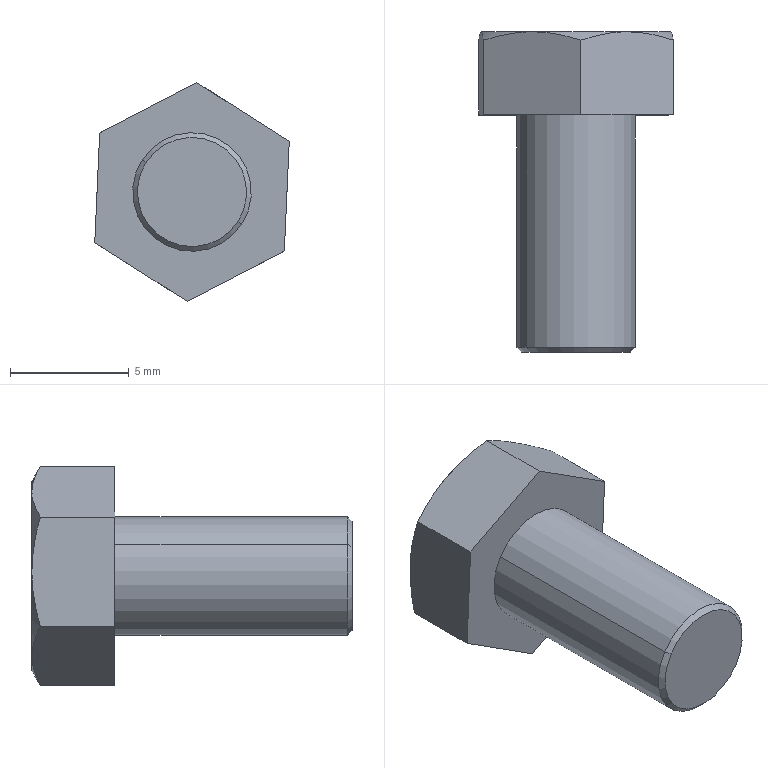Component | SolidWorks | TRCBASHexagonThroughHoleBolt[TRCBAS5-10]-1 | 1 solid | 20 faces | box 8.2 x 13.5 x 9.23 mm | volume 389 mm3 | cone 9 | plane 9 | cylinder 2 | commonest cylinder face diameters 5 x2
STEP:
#1=CARTESIAN_POINT('',(1.307,-10.008,-29.746));
#2=VERTEX_POINT('',#1);
#3=CARTESIAN_POINT('',(1.154,-10.008,-29.648));
#4=VERTEX_POINT('',#3);
#5=CARTESIAN_POINT('',(1.23,-10.008,-29.697));
#6=DIRECTION('',(0.,-1.,0.));
#7=DIRECTION('',(0.8429,0.,-0.5381));
#8=AXIS2_PLACEMENT_3D('',#5,#6,#7);
#9=CIRCLE('',#8,0.09055);
#10=EDGE_CURVE('',#2,#4,#9,.T.);
#11=ORIENTED_EDGE('',*,*,#10,.F.);
#12=CARTESIAN_POINT('',(1.313,-10.,-29.75));
#13=VERTEX_POINT('',#12);
#14=CARTESIAN_POINT('',(1.313,-10.,-29.75));
#15=DIRECTION('',(0.596,0.7071,-0.3805));
#16=VECTOR('',#15,39.37);
#17=LINE('',#14,#16);
#18=EDGE_CURVE('',#2,#13,#17,.T.);
#19=ORIENTED_EDGE('',*,*,#18,.T.);
#20=CARTESIAN_POINT('',(1.147,-10.,-29.644));
#21=VERTEX_POINT('',#20);
#22=CARTESIAN_POINT('',(1.23,-10.,-29.697));
#23=DIRECTION('',(-0.,1.,-0.));
#24=DIRECTION('',(0.8429,0.,-0.5381));
#25=AXIS2_PLACEMENT_3D('',#22,#23,#24);
#26=CIRCLE('',#25,0.09843);
#27=EDGE_CURVE('',#21,#13,#26,.T.);
#28=ORIENTED_EDGE('',*,*,#27,.F.);
#29=CARTESIAN_POINT('',(1.147,-10.,-29.644));
#30=DIRECTION('',(-0.596,0.7071,0.3805));
#31=VECTOR('',#30,39.37);
#32=LINE('',#29,#31);
#33=EDGE_CURVE('',#4,#21,#32,.T.);
#34=ORIENTED_EDGE('',*,*,#33,.F.);
#35=EDGE_LOOP('',(#11,#19,#28,#34));
#36=FACE_OUTER_BOUND('',#35,.T.);
#37=CARTESIAN_POINT('',(1.23,-10.,-29.697));
#38=DIRECTION('',(-0.,1.,-0.));
#39=DIRECTION('',(-0.8429,0.,0.5381));
#40=AXIS2_PLACEMENT_3D('',#37,#38,#39);
#41=CONICAL_SURFACE('',#40,0.09843,0.7854);
#42=ADVANCED_FACE('',(#36),#41,.T.);
#43=CARTESIAN_POINT('',(1.363,-9.477,-29.782));
#44=VERTEX_POINT('',#43);
#45=CARTESIAN_POINT('',(1.303,-9.477,-29.837));
#46=VERTEX_POINT('',#45);
#47=CARTESIAN_POINT('',(1.23,-9.477,-29.697));
#48=DIRECTION('',(-0.,1.,0.));
#49=DIRECTION('',(-0.8429,0.,0.5381));
#50=AXIS2_PLACEMENT_3D('',#47,#48,#49);
#51=CIRCLE('',#50,0.1575);
#52=EDGE_CURVE('',#44,#46,#51,.T.);
#53=ORIENTED_EDGE('',*,*,#52,.F.);
#54=CARTESIAN_POINT('',(1.384,-9.491,-29.795));
#55=VERTEX_POINT('',#54);
#56=CARTESIAN_POINT('',(1.363,-9.477,-29.782));
#57=DIRECTION('',(0.7299,-0.5,-0.466));
#58=VECTOR('',#57,39.37);
#59=LINE('',#56,#58);
#60=EDGE_CURVE('',#44,#55,#59,.T.);
#61=ORIENTED_EDGE('',*,*,#60,.T.);
#62=CARTESIAN_POINT('',(1.303,-9.477,-29.837));
#63=CARTESIAN_POINT('',(1.317,-9.477,-29.83));
#64=CARTESIAN_POINT('',(1.33,-9.478,-29.822));
#65=CARTESIAN_POINT('',(1.357,-9.483,-29.808));
#66=CARTESIAN_POINT('',(1.37,-9.486,-29.802));
#67=CARTESIAN_POINT('',(1.384,-9.491,-29.795));
#68=B_SPLINE_CURVE_WITH_KNOTS('',3,(#62,#63,#64,#65,#66,#67),.UNSPECIFIED.,.F.,.F.,(4,2,4),(0.002337,0.003501,0.004665),.UNSPECIFIED.);
#69=EDGE_CURVE('',#46,#55,#68,.T.);
#70=ORIENTED_EDGE('',*,*,#69,.F.);
#71=EDGE_LOOP('',(#53,#61,#70));
#72=FACE_OUTER_BOUND('',#71,.T.);
#73=CARTESIAN_POINT('',(1.23,-9.477,-29.697));
#74=DIRECTION('',(0.,-1.,0.));
#75=DIRECTION('',(0.8429,0.,-0.5381));
#76=AXIS2_PLACEMENT_3D('',#73,#74,#75);
#77=CONICAL_SURFACE('',#76,0.1575,1.047);
#78=ADVANCED_FACE('',(#72),#77,.T.);
#79=ORIENTED_EDGE('',*,*,#27,.T.);
#80=CARTESIAN_POINT('',(1.313,-9.614,-29.75));
#81=VERTEX_POINT('',#80);
#82=CARTESIAN_POINT('',(1.313,-9.477,-29.75));
#83=DIRECTION('',(-0.,1.,0.));
#84=VECTOR('',#83,39.37);
#85=LINE('',#82,#84);
#86=EDGE_CURVE('',#13,#81,#85,.T.);
#87=ORIENTED_EDGE('',*,*,#86,.T.);
#88=CARTESIAN_POINT('',(1.147,-9.614,-29.644));
#89=VERTEX_POINT('',#88);
#90=CARTESIAN_POINT('',(1.23,-9.614,-29.697));
#91=DIRECTION('',(-0.,1.,0.));
#92=DIRECTION('',(-0.8429,0.,0.5381));
#93=AXIS2_PLACEMENT_3D('',#90,#91,#92);
#94=CIRCLE('',#93,0.09843);
#95=EDGE_CURVE('',#89,#81,#94,.T.);
#96=ORIENTED_EDGE('',*,*,#95,.F.);
#97=CARTESIAN_POINT('',(1.147,-9.477,-29.644));
#98=DIRECTION('',(-0.,1.,0.));
#99=VECTOR('',#98,39.37);
#100=LINE('',#97,#99);
#101=EDGE_CURVE('',#21,#89,#100,.T.);
#102=ORIENTED_EDGE('',*,*,#101,.F.);
#103=EDGE_LOOP('',(#79,#87,#96,#102));
#104=FACE_OUTER_BOUND('',#103,.T.);
#105=CARTESIAN_POINT('',(1.23,-9.477,-29.697));
#106=DIRECTION('',(-0.,1.,0.));
#107=DIRECTION('',(-0.8429,0.,0.5381));
#108=AXIS2_PLACEMENT_3D('',#105,#106,#107);
#109=CYLINDRICAL_SURFACE('',#108,0.09843);
#110=ADVANCED_FACE('',(#104),#109,.T.);
#111=CARTESIAN_POINT('',(1.384,-9.614,-29.795));
#112=VERTEX_POINT('',#111);
#113=CARTESIAN_POINT('',(1.384,-9.614,-29.795));
#114=DIRECTION('',(-0.,1.,-0.));
#115=VECTOR('',#114,39.37);
#116=LINE('',#113,#115);
#117=EDGE_CURVE('',#112,#55,#116,.T.);
#118=ORIENTED_EDGE('',*,*,#117,.T.);
#119=CARTESIAN_POINT('',(1.388,-9.477,-29.704));
#120=VERTEX_POINT('',#119);
#121=CARTESIAN_POINT('',(1.384,-9.491,-29.795));
#122=CARTESIAN_POINT('',(1.385,-9.482,-29.765));
#123=CARTESIAN_POINT('',(1.386,-9.477,-29.735));
#124=CARTESIAN_POINT('',(1.388,-9.477,-29.704));
#125=B_SPLINE_CURVE_WITH_KNOTS('',3,(#121,#122,#123,#124),.UNSPECIFIED.,.F.,.F.,(4,4),(0.00000024,0.002337),.UNSPECIFIED.);
#126=EDGE_CURVE('',#55,#120,#125,.T.);
#127=ORIENTED_EDGE('',*,*,#126,.T.);
#128=CARTESIAN_POINT('',(1.392,-9.491,-29.613));
#129=VERTEX_POINT('',#128);
#130=CARTESIAN_POINT('',(1.388,-9.477,-29.704));
#131=CARTESIAN_POINT('',(1.388,-9.477,-29.688));
#132=CARTESIAN_POINT('',(1.389,-9.478,-29.673));
#133=CARTESIAN_POINT('',(1.39,-9.483,-29.643));
#134=CARTESIAN_POINT('',(1.391,-9.486,-29.628));
#135=CARTESIAN_POINT('',(1.392,-9.491,-29.613));
#136=B_SPLINE_CURVE_WITH_KNOTS('',3,(#130,#131,#132,#133,#134,#135),.UNSPECIFIED.,.F.,.F.,(4,2,4),(0.002337,0.003501,0.004665),.UNSPECIFIED.);
#137=EDGE_CURVE('',#120,#129,#136,.T.);
#138=ORIENTED_EDGE('',*,*,#137,.T.);
#139=CARTESIAN_POINT('',(1.392,-9.614,-29.613));
#140=VERTEX_POINT('',#139);
#141=CARTESIAN_POINT('',(1.392,-9.614,-29.613));
#142=DIRECTION('',(-0.,1.,-0.));
#143=VECTOR('',#142,39.37);
#144=LINE('',#141,#143);
#145=EDGE_CURVE('',#140,#129,#144,.T.);
#146=ORIENTED_EDGE('',*,*,#145,.F.);
#147=CARTESIAN_POINT('',(1.392,-9.614,-29.613));
#148=DIRECTION('',(-0.04461,-0.,-0.999));
#149=VECTOR('',#148,39.37);
#150=LINE('',#147,#149);
#151=EDGE_CURVE('',#140,#112,#150,.T.);
#152=ORIENTED_EDGE('',*,*,#151,.T.);
#153=EDGE_LOOP('',(#118,#127,#138,#146,#152));
#154=FACE_OUTER_BOUND('',#153,.T.);
#155=CARTESIAN_POINT('',(1.392,-9.614,-29.613));
#156=DIRECTION('',(0.999,0.,-0.04461));
#157=DIRECTION('',(-0.04461,-0.,-0.999));
#158=AXIS2_PLACEMENT_3D('',#155,#156,#157);
#159=PLANE('',#158);
#160=ADVANCED_FACE('',(#154),#159,.T.);
#161=ORIENTED_EDGE('',*,*,#145,.T.);
#162=CARTESIAN_POINT('',(1.315,-9.477,-29.564));
#163=VERTEX_POINT('',#162);
#164=CARTESIAN_POINT('',(1.392,-9.491,-29.613));
#165=CARTESIAN_POINT('',(1.379,-9.486,-29.605));
#166=CARTESIAN_POINT('',(1.367,-9.483,-29.597));
#167=CARTESIAN_POINT('',(1.341,-9.478,-29.581));
#168=CARTESIAN_POINT('',(1.328,-9.477,-29.572));
#169=CARTESIAN_POINT('',(1.315,-9.477,-29.564));
#170=B_SPLINE_CURVE_WITH_KNOTS('',3,(#164,#165,#166,#167,#168,#169),.UNSPECIFIED.,.F.,.F.,(4,2,4),(0.01187,0.01304,0.01421),.UNSPECIFIED.);
#171=EDGE_CURVE('',#129,#163,#170,.T.);
#172=ORIENTED_EDGE('',*,*,#171,.T.);
#173=CARTESIAN_POINT('',(1.238,-9.491,-29.515));
#174=VERTEX_POINT('',#173);
#175=CARTESIAN_POINT('',(1.315,-9.477,-29.564));
#176=CARTESIAN_POINT('',(1.302,-9.477,-29.556));
#177=CARTESIAN_POINT('',(1.289,-9.478,-29.548));
#178=CARTESIAN_POINT('',(1.264,-9.483,-29.531));
#179=CARTESIAN_POINT('',(1.251,-9.486,-29.523));
#180=CARTESIAN_POINT('',(1.238,-9.491,-29.515));
#181=B_SPLINE_CURVE_WITH_KNOTS('',3,(#175,#176,#177,#178,#179,#180),.UNSPECIFIED.,.F.,.F.,(4,2,4),(0.01421,0.01538,0.01654),.UNSPECIFIED.);
#182=EDGE_CURVE('',#163,#174,#181,.T.);
#183=ORIENTED_EDGE('',*,*,#182,.T.);
#184=CARTESIAN_POINT('',(1.238,-9.614,-29.515));
#185=VERTEX_POINT('',#184);
#186=CARTESIAN_POINT('',(1.238,-9.614,-29.515));
#187=DIRECTION('',(-0.,1.,-0.));
#188=VECTOR('',#187,39.37);
#189=LINE('',#186,#188);
#190=EDGE_CURVE('',#185,#174,#189,.T.);
#191=ORIENTED_EDGE('',*,*,#190,.F.);
#192=CARTESIAN_POINT('',(1.238,-9.614,-29.515));
#193=DIRECTION('',(0.8429,0.,-0.5381));
#194=VECTOR('',#193,39.37);
#195=LINE('',#192,#194);
#196=EDGE_CURVE('',#185,#140,#195,.T.);
#197=ORIENTED_EDGE('',*,*,#196,.T.);
#198=EDGE_LOOP('',(#161,#172,#183,#191,#197));
#199=FACE_OUTER_BOUND('',#198,.T.);
#200=CARTESIAN_POINT('',(1.238,-9.614,-29.515));
#201=DIRECTION('',(0.5381,0.,0.8429));
#202=DIRECTION('',(0.8429,0.,-0.5381));
#203=AXIS2_PLACEMENT_3D('',#200,#201,#202);
#204=PLANE('',#203);
#205=ADVANCED_FACE('',(#199),#204,.T.);
#206=ORIENTED_EDGE('',*,*,#190,.T.);
#207=CARTESIAN_POINT('',(1.158,-9.477,-29.557));
#208=VERTEX_POINT('',#207);
#209=CARTESIAN_POINT('',(1.238,-9.491,-29.515));
#210=CARTESIAN_POINT('',(1.212,-9.482,-29.529));
#211=CARTESIAN_POINT('',(1.185,-9.477,-29.543));
#212=CARTESIAN_POINT('',(1.158,-9.477,-29.557));
#213=B_SPLINE_CURVE_WITH_KNOTS('',3,(#209,#210,#211,#212),.UNSPECIFIED.,.F.,.F.,(4,4),(0.00000024,0.002337),.UNSPECIFIED.);
#214=EDGE_CURVE('',#174,#208,#213,.T.);
#215=ORIENTED_EDGE('',*,*,#214,.T.);
#216=CARTESIAN_POINT('',(1.077,-9.491,-29.599));
#217=VERTEX_POINT('',#216);
#218=CARTESIAN_POINT('',(1.158,-9.477,-29.557));
#219=CARTESIAN_POINT('',(1.144,-9.477,-29.564));
#220=CARTESIAN_POINT('',(1.13,-9.478,-29.571));
#221=CARTESIAN_POINT('',(1.103,-9.483,-29.585));
#222=CARTESIAN_POINT('',(1.09,-9.486,-29.592));
#223=CARTESIAN_POINT('',(1.077,-9.491,-29.599));
#224=B_SPLINE_CURVE_WITH_KNOTS('',3,(#218,#219,#220,#221,#222,#223),.UNSPECIFIED.,.F.,.F.,(4,2,4),(0.002337,0.003501,0.004665),.UNSPECIFIED.);
#225=EDGE_CURVE('',#208,#217,#224,.T.);
#226=ORIENTED_EDGE('',*,*,#225,.T.);
#227=CARTESIAN_POINT('',(1.077,-9.614,-29.599));
#228=VERTEX_POINT('',#227);
#229=CARTESIAN_POINT('',(1.077,-9.614,-29.599));
#230=DIRECTION('',(-0.,1.,-0.));
#231=VECTOR('',#230,39.37);
#232=LINE('',#229,#231);
#233=EDGE_CURVE('',#228,#217,#232,.T.);
#234=ORIENTED_EDGE('',*,*,#233,.F.);
#235=CARTESIAN_POINT('',(1.077,-9.614,-29.599));
#236=DIRECTION('',(0.8875,0.,0.4609));
#237=VECTOR('',#236,39.37);
#238=LINE('',#235,#237);
#239=EDGE_CURVE('',#228,#185,#238,.T.);
#240=ORIENTED_EDGE('',*,*,#239,.T.);
#241=EDGE_LOOP('',(#206,#215,#226,#234,#240));
#242=FACE_OUTER_BOUND('',#241,.T.);
#243=CARTESIAN_POINT('',(1.077,-9.614,-29.599));
#244=DIRECTION('',(-0.4609,-0.,0.8875));
#245=DIRECTION('',(0.8875,0.,0.4609));
#246=AXIS2_PLACEMENT_3D('',#243,#244,#245);
#247=PLANE('',#246);
#248=ADVANCED_FACE('',(#242),#247,.T.);
#249=ORIENTED_EDGE('',*,*,#233,.T.);
#250=CARTESIAN_POINT('',(1.073,-9.477,-29.69));
#251=VERTEX_POINT('',#250);
#252=CARTESIAN_POINT('',(1.077,-9.491,-29.599));
#253=CARTESIAN_POINT('',(1.076,-9.482,-29.629));
#254=CARTESIAN_POINT('',(1.074,-9.477,-29.659));
#255=CARTESIAN_POINT('',(1.073,-9.477,-29.69));
#256=B_SPLINE_CURVE_WITH_KNOTS('',3,(#252,#253,#254,#255),.UNSPECIFIED.,.F.,.F.,(4,4),(0.00000024,0.002337),.UNSPECIFIED.);
#257=EDGE_CURVE('',#217,#251,#256,.T.);
#258=ORIENTED_EDGE('',*,*,#257,.T.);
#259=CARTESIAN_POINT('',(1.069,-9.491,-29.781));
#260=VERTEX_POINT('',#259);
#261=CARTESIAN_POINT('',(1.073,-9.477,-29.69));
#262=CARTESIAN_POINT('',(1.072,-9.477,-29.705));
#263=CARTESIAN_POINT('',(1.072,-9.478,-29.721));
#264=CARTESIAN_POINT('',(1.07,-9.483,-29.751));
#265=CARTESIAN_POINT('',(1.07,-9.486,-29.766));
#266=CARTESIAN_POINT('',(1.069,-9.491,-29.781));
#267=B_SPLINE_CURVE_WITH_KNOTS('',3,(#261,#262,#263,#264,#265,#266),.UNSPECIFIED.,.F.,.F.,(4,2,4),(0.002337,0.003501,0.004665),.UNSPECIFIED.);
#268=EDGE_CURVE('',#251,#260,#267,.T.);
#269=ORIENTED_EDGE('',*,*,#268,.T.);
#270=CARTESIAN_POINT('',(1.069,-9.614,-29.781));
#271=VERTEX_POINT('',#270);
#272=CARTESIAN_POINT('',(1.069,-9.614,-29.781));
#273=DIRECTION('',(-0.,1.,-0.));
#274=VECTOR('',#273,39.37);
#275=LINE('',#272,#274);
#276=EDGE_CURVE('',#271,#260,#275,.T.);
#277=ORIENTED_EDGE('',*,*,#276,.F.);
#278=CARTESIAN_POINT('',(1.069,-9.614,-29.781));
#279=DIRECTION('',(0.04461,0.,0.999));
#280=VECTOR('',#279,39.37);
#281=LINE('',#278,#280);
#282=EDGE_CURVE('',#271,#228,#281,.T.);
#283=ORIENTED_EDGE('',*,*,#282,.T.);
#284=EDGE_LOOP('',(#249,#258,#269,#277,#283));
#285=FACE_OUTER_BOUND('',#284,.T.);
#286=CARTESIAN_POINT('',(1.069,-9.614,-29.781));
#287=DIRECTION('',(-0.999,-0.,0.04461));
#288=DIRECTION('',(0.04461,0.,0.999));
#289=AXIS2_PLACEMENT_3D('',#286,#287,#288);
#290=PLANE('',#289);
#291=ADVANCED_FACE('',(#285),#290,.T.);
#292=ORIENTED_EDGE('',*,*,#276,.T.);
#293=CARTESIAN_POINT('',(1.146,-9.477,-29.83));
#294=VERTEX_POINT('',#293);
#295=CARTESIAN_POINT('',(1.069,-9.491,-29.781));
#296=CARTESIAN_POINT('',(1.081,-9.486,-29.789));
#297=CARTESIAN_POINT('',(1.094,-9.483,-29.797));
#298=CARTESIAN_POINT('',(1.12,-9.478,-29.813));
#299=CARTESIAN_POINT('',(1.133,-9.477,-29.821));
#300=CARTESIAN_POINT('',(1.146,-9.477,-29.83));
#301=B_SPLINE_CURVE_WITH_KNOTS('',3,(#295,#296,#297,#298,#299,#300),.UNSPECIFIED.,.F.,.F.,(4,2,4),(0.004244,0.005413,0.006581),.UNSPECIFIED.);
#302=EDGE_CURVE('',#260,#294,#301,.T.);
#303=ORIENTED_EDGE('',*,*,#302,.T.);
#304=CARTESIAN_POINT('',(1.222,-9.491,-29.879));
#305=VERTEX_POINT('',#304);
#306=CARTESIAN_POINT('',(1.146,-9.477,-29.83));
#307=CARTESIAN_POINT('',(1.159,-9.477,-29.838));
#308=CARTESIAN_POINT('',(1.172,-9.478,-29.846));
#309=CARTESIAN_POINT('',(1.197,-9.483,-29.863));
#310=CARTESIAN_POINT('',(1.21,-9.486,-29.871));
#311=CARTESIAN_POINT('',(1.222,-9.491,-29.879));
#312=B_SPLINE_CURVE_WITH_KNOTS('',3,(#306,#307,#308,#309,#310,#311),.UNSPECIFIED.,.F.,.F.,(4,2,4),(0.006581,0.007751,0.008921),.UNSPECIFIED.);
#313=EDGE_CURVE('',#294,#305,#312,.T.);
#314=ORIENTED_EDGE('',*,*,#313,.T.);
#315=CARTESIAN_POINT('',(1.222,-9.614,-29.879));
#316=VERTEX_POINT('',#315);
#317=CARTESIAN_POINT('',(1.222,-9.614,-29.879));
#318=DIRECTION('',(-0.,1.,-0.));
#319=VECTOR('',#318,39.37);
#320=LINE('',#317,#319);
#321=EDGE_CURVE('',#316,#305,#320,.T.);
#322=ORIENTED_EDGE('',*,*,#321,.F.);
#323=CARTESIAN_POINT('',(1.222,-9.614,-29.879));
#324=DIRECTION('',(-0.8429,-0.,0.5381));
#325=VECTOR('',#324,39.37);
#326=LINE('',#323,#325);
#327=EDGE_CURVE('',#316,#271,#326,.T.);
#328=ORIENTED_EDGE('',*,*,#327,.T.);
#329=EDGE_LOOP('',(#292,#303,#314,#322,#328));
#330=FACE_OUTER_BOUND('',#329,.T.);
#331=CARTESIAN_POINT('',(1.222,-9.614,-29.879));
#332=DIRECTION('',(-0.5381,-0.,-0.8429));
#333=DIRECTION('',(-0.8429,-0.,0.5381));
#334=AXIS2_PLACEMENT_3D('',#331,#332,#333);
#335=PLANE('',#334);
#336=ADVANCED_FACE('',(#330),#335,.T.);
#337=ORIENTED_EDGE('',*,*,#321,.T.);
#338=CARTESIAN_POINT('',(1.222,-9.491,-29.879));
#339=CARTESIAN_POINT('',(1.249,-9.482,-29.865));
#340=CARTESIAN_POINT('',(1.275,-9.477,-29.851));
#341=CARTESIAN_POINT('',(1.303,-9.477,-29.837));
#342=B_SPLINE_CURVE_WITH_KNOTS('',3,(#338,#339,#340,#341),.UNSPECIFIED.,.F.,.F.,(4,4),(0.00000024,0.002337),.UNSPECIFIED.);
#343=EDGE_CURVE('',#305,#46,#342,.T.);
#344=ORIENTED_EDGE('',*,*,#343,.T.);
#345=ORIENTED_EDGE('',*,*,#69,.T.);
#346=ORIENTED_EDGE('',*,*,#117,.F.);
#347=CARTESIAN_POINT('',(1.384,-9.614,-29.795));
#348=DIRECTION('',(-0.8875,-0.,-0.4609));
#349=VECTOR('',#348,39.37);
#350=LINE('',#347,#349);
#351=EDGE_CURVE('',#112,#316,#350,.T.);
#352=ORIENTED_EDGE('',*,*,#351,.T.);
#353=EDGE_LOOP('',(#337,#344,#345,#346,#352));
#354=FACE_OUTER_BOUND('',#353,.T.);
#355=CARTESIAN_POINT('',(1.384,-9.614,-29.795));
#356=DIRECTION('',(0.4609,0.,-0.8875));
#357=DIRECTION('',(-0.8875,-0.,-0.4609));
#358=AXIS2_PLACEMENT_3D('',#355,#356,#357);
#359=PLANE('',#358);
#360=ADVANCED_FACE('',(#354),#359,.T.);
#361=ORIENTED_EDGE('',*,*,#95,.T.);
#362=CARTESIAN_POINT('',(1.23,-9.614,-29.697));
#363=DIRECTION('',(-0.,1.,0.));
#364=DIRECTION('',(-0.8429,0.,0.5381));
#365=AXIS2_PLACEMENT_3D('',#362,#363,#364);
#366=CIRCLE('',#365,0.09843);
#367=EDGE_CURVE('',#81,#89,#366,.T.);
#368=ORIENTED_EDGE('',*,*,#367,.T.);
#369=EDGE_LOOP('',(#361,#368));
#370=FACE_BOUND('',#369,.T.);
#371=ORIENTED_EDGE('',*,*,#239,.F.);
#372=ORIENTED_EDGE('',*,*,#282,.F.);
#373=ORIENTED_EDGE('',*,*,#327,.F.);
#374=ORIENTED_EDGE('',*,*,#351,.F.);
#375=ORIENTED_EDGE('',*,*,#151,.F.);
#376=ORIENTED_EDGE('',*,*,#196,.F.);
#377=EDGE_LOOP('',(#371,#372,#373,#374,#375,#376));
#378=FACE_OUTER_BOUND('',#377,.T.);
#379=CARTESIAN_POINT('',(1.363,-9.614,-29.782));
#380=DIRECTION('',(0.,-1.,0.));
#381=DIRECTION('',(0.8429,0.,-0.5381));
#382=AXIS2_PLACEMENT_3D('',#379,#380,#381);
#383=PLANE('',#382);
#384=ADVANCED_FACE('',(#370,#378),#383,.T.);
#385=ORIENTED_EDGE('',*,*,#86,.F.);
#386=CARTESIAN_POINT('',(1.23,-10.,-29.697));
#387=DIRECTION('',(-0.,1.,-0.));
#388=DIRECTION('',(0.8429,0.,-0.5381));
#389=AXIS2_PLACEMENT_3D('',#386,#387,#388);
#390=CIRCLE('',#389,0.09843);
#391=EDGE_CURVE('',#13,#21,#390,.T.);
#392=ORIENTED_EDGE('',*,*,#391,.T.);
#393=ORIENTED_EDGE('',*,*,#101,.T.);
#394=ORIENTED_EDGE('',*,*,#367,.F.);
#395=EDGE_LOOP('',(#385,#392,#393,#394));
#396=FACE_OUTER_BOUND('',#395,.T.);
#397=CARTESIAN_POINT('',(1.23,-9.477,-29.697));
#398=DIRECTION('',(-0.,1.,0.));
#399=DIRECTION('',(-0.8429,0.,0.5381));
#400=AXIS2_PLACEMENT_3D('',#397,#398,#399);
#401=CYLINDRICAL_SURFACE('',#400,0.09843);
#402=ADVANCED_FACE('',(#396),#401,.T.);
#403=CARTESIAN_POINT('',(1.23,-10.008,-29.697));
#404=DIRECTION('',(0.,-1.,0.));
#405=DIRECTION('',(0.8429,0.,-0.5381));
#406=AXIS2_PLACEMENT_3D('',#403,#404,#405);
#407=CIRCLE('',#406,0.09055);
#408=EDGE_CURVE('',#4,#2,#407,.T.);
#409=ORIENTED_EDGE('',*,*,#408,.T.);
#410=ORIENTED_EDGE('',*,*,#10,.T.);
#411=EDGE_LOOP('',(#409,#410));
#412=FACE_OUTER_BOUND('',#411,.T.);
#413=CARTESIAN_POINT('',(1.313,-10.008,-29.75));
#414=DIRECTION('',(0.,-1.,0.));
#415=DIRECTION('',(0.8429,0.,-0.5381));
#416=AXIS2_PLACEMENT_3D('',#413,#414,#415);
#417=PLANE('',#416);
#418=ADVANCED_FACE('',(#412),#417,.T.);
#419=CARTESIAN_POINT('',(1.23,-9.477,-29.697));
#420=DIRECTION('',(-0.,1.,0.));
#421=DIRECTION('',(-0.8429,0.,0.5381));
#422=AXIS2_PLACEMENT_3D('',#419,#420,#421);
#423=CIRCLE('',#422,0.1575);
#424=EDGE_CURVE('',#251,#208,#423,.T.);
#425=ORIENTED_EDGE('',*,*,#424,.F.);
#426=ORIENTED_EDGE('',*,*,#257,.F.);
#427=ORIENTED_EDGE('',*,*,#225,.F.);
#428=EDGE_LOOP('',(#425,#426,#427));
#429=FACE_OUTER_BOUND('',#428,.T.);
#430=CARTESIAN_POINT('',(1.23,-9.477,-29.697));
#431=DIRECTION('',(0.,-1.,0.));
#432=DIRECTION('',(0.8429,0.,-0.5381));
#433=AXIS2_PLACEMENT_3D('',#430,#431,#432);
#434=CONICAL_SURFACE('',#433,0.1575,1.047);
#435=ADVANCED_FACE('',(#429),#434,.T.);
#436=CARTESIAN_POINT('',(1.23,-9.477,-29.697));
#437=DIRECTION('',(-0.,1.,0.));
#438=DIRECTION('',(-0.8429,0.,0.5381));
#439=AXIS2_PLACEMENT_3D('',#436,#437,#438);
#440=CIRCLE('',#439,0.1575);
#441=EDGE_CURVE('',#294,#251,#440,.T.);
#442=ORIENTED_EDGE('',*,*,#441,.F.);
#443=ORIENTED_EDGE('',*,*,#302,.F.);
#444=ORIENTED_EDGE('',*,*,#268,.F.);
#445=EDGE_LOOP('',(#442,#443,#444));
#446=FACE_OUTER_BOUND('',#445,.T.);
#447=CARTESIAN_POINT('',(1.23,-9.477,-29.697));
#448=DIRECTION('',(0.,-1.,0.));
#449=DIRECTION('',(0.8429,0.,-0.5381));
#450=AXIS2_PLACEMENT_3D('',#447,#448,#449);
#451=CONICAL_SURFACE('',#450,0.1575,1.047);
#452=ADVANCED_FACE('',(#446),#451,.T.);
#453=CARTESIAN_POINT('',(1.23,-9.477,-29.697));
#454=DIRECTION('',(-0.,1.,0.));
#455=DIRECTION('',(-0.8429,0.,0.5381));
#456=AXIS2_PLACEMENT_3D('',#453,#454,#455);
#457=CIRCLE('',#456,0.1575);
#458=EDGE_CURVE('',#46,#294,#457,.T.);
#459=ORIENTED_EDGE('',*,*,#458,.F.);
#460=ORIENTED_EDGE('',*,*,#343,.F.);
#461=ORIENTED_EDGE('',*,*,#313,.F.);
#462=EDGE_LOOP('',(#459,#460,#461));
#463=FACE_OUTER_BOUND('',#462,.T.);
#464=CARTESIAN_POINT('',(1.23,-9.477,-29.697));
#465=DIRECTION('',(0.,-1.,0.));
#466=DIRECTION('',(0.8429,0.,-0.5381));
#467=AXIS2_PLACEMENT_3D('',#464,#465,#466);
#468=CONICAL_SURFACE('',#467,0.1575,1.047);
#469=ADVANCED_FACE('',(#463),#468,.T.);
#470=ORIENTED_EDGE('',*,*,#60,.F.);
#471=CARTESIAN_POINT('',(1.23,-9.477,-29.697));
#472=DIRECTION('',(-0.,1.,0.));
#473=DIRECTION('',(-0.8429,0.,0.5381));
#474=AXIS2_PLACEMENT_3D('',#471,#472,#473);
#475=CIRCLE('',#474,0.1575);
#476=EDGE_CURVE('',#120,#44,#475,.T.);
#477=ORIENTED_EDGE('',*,*,#476,.F.);
#478=ORIENTED_EDGE('',*,*,#126,.F.);
#479=EDGE_LOOP('',(#470,#477,#478));
#480=FACE_OUTER_BOUND('',#479,.T.);
#481=CARTESIAN_POINT('',(1.23,-9.477,-29.697));
#482=DIRECTION('',(0.,-1.,0.));
#483=DIRECTION('',(0.8429,0.,-0.5381));
#484=AXIS2_PLACEMENT_3D('',#481,#482,#483);
#485=CONICAL_SURFACE('',#484,0.1575,1.047);
#486=ADVANCED_FACE('',(#480),#485,.T.);
#487=CARTESIAN_POINT('',(1.23,-9.477,-29.697));
#488=DIRECTION('',(-0.,1.,0.));
#489=DIRECTION('',(-0.8429,0.,0.5381));
#490=AXIS2_PLACEMENT_3D('',#487,#488,#489);
#491=CIRCLE('',#490,0.1575);
#492=EDGE_CURVE('',#163,#120,#491,.T.);
#493=ORIENTED_EDGE('',*,*,#492,.F.);
#494=ORIENTED_EDGE('',*,*,#171,.F.);
#495=ORIENTED_EDGE('',*,*,#137,.F.);
#496=EDGE_LOOP('',(#493,#494,#495));
#497=FACE_OUTER_BOUND('',#496,.T.);
#498=CARTESIAN_POINT('',(1.23,-9.477,-29.697));
#499=DIRECTION('',(0.,-1.,0.));
#500=DIRECTION('',(0.8429,0.,-0.5381));
#501=AXIS2_PLACEMENT_3D('',#498,#499,#500);
#502=CONICAL_SURFACE('',#501,0.1575,1.047);
#503=ADVANCED_FACE('',(#497),#502,.T.);
#504=CARTESIAN_POINT('',(1.23,-9.477,-29.697));
#505=DIRECTION('',(-0.,1.,0.));
#506=DIRECTION('',(-0.8429,0.,0.5381));
#507=AXIS2_PLACEMENT_3D('',#504,#505,#506);
#508=CIRCLE('',#507,0.1575);
#509=EDGE_CURVE('',#208,#163,#508,.T.);
#510=ORIENTED_EDGE('',*,*,#509,.F.);
#511=ORIENTED_EDGE('',*,*,#214,.F.);
#512=ORIENTED_EDGE('',*,*,#182,.F.);
#513=EDGE_LOOP('',(#510,#511,#512));
#514=FACE_OUTER_BOUND('',#513,.T.);
#515=CARTESIAN_POINT('',(1.23,-9.477,-29.697));
#516=DIRECTION('',(0.,-1.,0.));
#517=DIRECTION('',(0.8429,0.,-0.5381));
#518=AXIS2_PLACEMENT_3D('',#515,#516,#517);
#519=CONICAL_SURFACE('',#518,0.1575,1.047);
#520=ADVANCED_FACE('',(#514),#519,.T.);
#521=ORIENTED_EDGE('',*,*,#424,.T.);
#522=ORIENTED_EDGE('',*,*,#509,.T.);
#523=ORIENTED_EDGE('',*,*,#492,.T.);
#524=ORIENTED_EDGE('',*,*,#476,.T.);
#525=ORIENTED_EDGE('',*,*,#52,.T.);
#526=ORIENTED_EDGE('',*,*,#458,.T.);
#527=ORIENTED_EDGE('',*,*,#441,.T.);
#528=EDGE_LOOP('',(#521,#522,#523,#524,#525,#526,#527));
#529=FACE_OUTER_BOUND('',#528,.T.);
#530=CARTESIAN_POINT('',(1.363,-9.477,-29.782));
#531=DIRECTION('',(-0.,1.,-0.));
#532=DIRECTION('',(-0.8429,-0.,0.5381));
#533=AXIS2_PLACEMENT_3D('',#530,#531,#532);
#534=PLANE('',#533);
#535=ADVANCED_FACE('',(#529),#534,.T.);
#536=ORIENTED_EDGE('',*,*,#18,.F.);
#537=ORIENTED_EDGE('',*,*,#408,.F.);
#538=ORIENTED_EDGE('',*,*,#33,.T.);
#539=ORIENTED_EDGE('',*,*,#391,.F.);
#540=EDGE_LOOP('',(#536,#537,#538,#539));
#541=FACE_OUTER_BOUND('',#540,.T.);
#542=CARTESIAN_POINT('',(1.23,-10.,-29.697));
#543=DIRECTION('',(-0.,1.,-0.));
#544=DIRECTION('',(-0.8429,0.,0.5381));
#545=AXIS2_PLACEMENT_3D('',#542,#543,#544);
#546=CONICAL_SURFACE('',#545,0.09843,0.7854);
#547=ADVANCED_FACE('',(#541),#546,.T.);
#548=CLOSED_SHELL('',(#42,#78,#110,#160,#205,#248,#291,#336,#360,#384,#402,#418,#435,#452,#469,#486,#503,#520,#535,#547));
#549=MANIFOLD_SOLID_BREP('',#548);
#550=CARTESIAN_POINT('',(0.,0.,0.));
#551=DIRECTION('',(0.,0.,1.));
#552=DIRECTION('',(1.,0.,0.));
#553=AXIS2_PLACEMENT_3D('',#550,#551,#552);
#554=(LENGTH_UNIT()NAMED_UNIT(*)SI_UNIT($,.METRE.));
#555=LENGTH_MEASURE_WITH_UNIT(LENGTH_MEASURE(0.0254),#554);
#556=DIMENSIONAL_EXPONENTS(1.,0.,0.,0.,0.,0.,0.);
#557=(CONVERSION_BASED_UNIT('',#555)LENGTH_UNIT()NAMED_UNIT(#556));
#558=UNCERTAINTY_MEASURE_WITH_UNIT(LENGTH_MEASURE(0.00001),#557,'','');
#559=(NAMED_UNIT(*)PLANE_ANGLE_UNIT()SI_UNIT($,.RADIAN.));
#560=(NAMED_UNIT(*)SI_UNIT($,.STERADIAN.)SOLID_ANGLE_UNIT());
#561=(GEOMETRIC_REPRESENTATION_CONTEXT(3)GLOBAL_UNCERTAINTY_ASSIGNED_CONTEXT((#558))GLOBAL_UNIT_ASSIGNED_CONTEXT((#557,#559,#560))REPRESENTATION_CONTEXT('',''));
#562=ADVANCED_BREP_SHAPE_REPRESENTATION('',(#549,#553),#561);
#563=COLOUR_RGB('',0.7922,0.8196,0.9333);
#564=FILL_AREA_STYLE_COLOUR('',#563);
#565=FILL_AREA_STYLE('',(#564));
#566=SURFACE_STYLE_FILL_AREA(#565);
#567=SURFACE_SIDE_STYLE('',(#566));
#568=SURFACE_STYLE_USAGE(.BOTH.,#567);
#569=PRESENTATION_STYLE_ASSIGNMENT((#568));
#570=STYLED_ITEM('',(#569),#549);
#571=PRESENTATION_LAYER_ASSIGNMENT('','',(#570));
#572=(LENGTH_UNIT()NAMED_UNIT(*)SI_UNIT($,.METRE.));
#573=LENGTH_MEASURE_WITH_UNIT(LENGTH_MEASURE(0.0254),#572);
#574=DIMENSIONAL_EXPONENTS(1.,0.,0.,0.,0.,0.,0.);
#575=(CONVERSION_BASED_UNIT('',#573)LENGTH_UNIT()NAMED_UNIT(#574));
#576=UNCERTAINTY_MEASURE_WITH_UNIT(LENGTH_MEASURE(0.00001),#575,'','');
#577=(NAMED_UNIT(*)PLANE_ANGLE_UNIT()SI_UNIT($,.RADIAN.));
#578=(NAMED_UNIT(*)SI_UNIT($,.STERADIAN.)SOLID_ANGLE_UNIT());
#579=(GEOMETRIC_REPRESENTATION_CONTEXT(3)GLOBAL_UNCERTAINTY_ASSIGNED_CONTEXT((#576))GLOBAL_UNIT_ASSIGNED_CONTEXT((#575,#577,#578))REPRESENTATION_CONTEXT('',''));
#580=MECHANICAL_DESIGN_GEOMETRIC_PRESENTATION_REPRESENTATION('',(#570),#579);